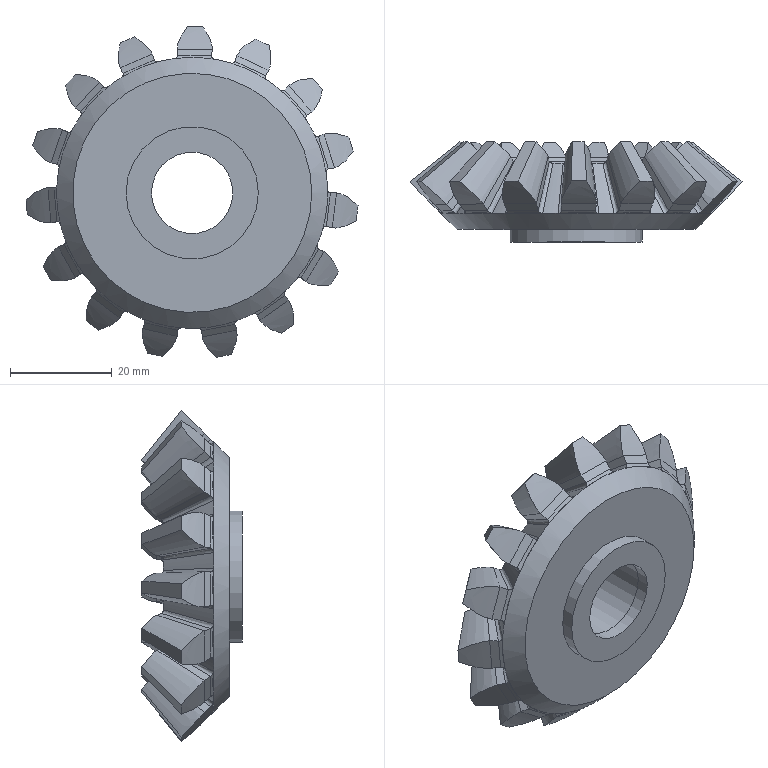Component | NX | BEVEL_GEAR_1 | 2 solids | 249 faces | volume 25150 mm3 | spline 150 | plane 64 | cone 32 | cylinder 3 | commonest cylinder face diameters 16 x2 26 x1